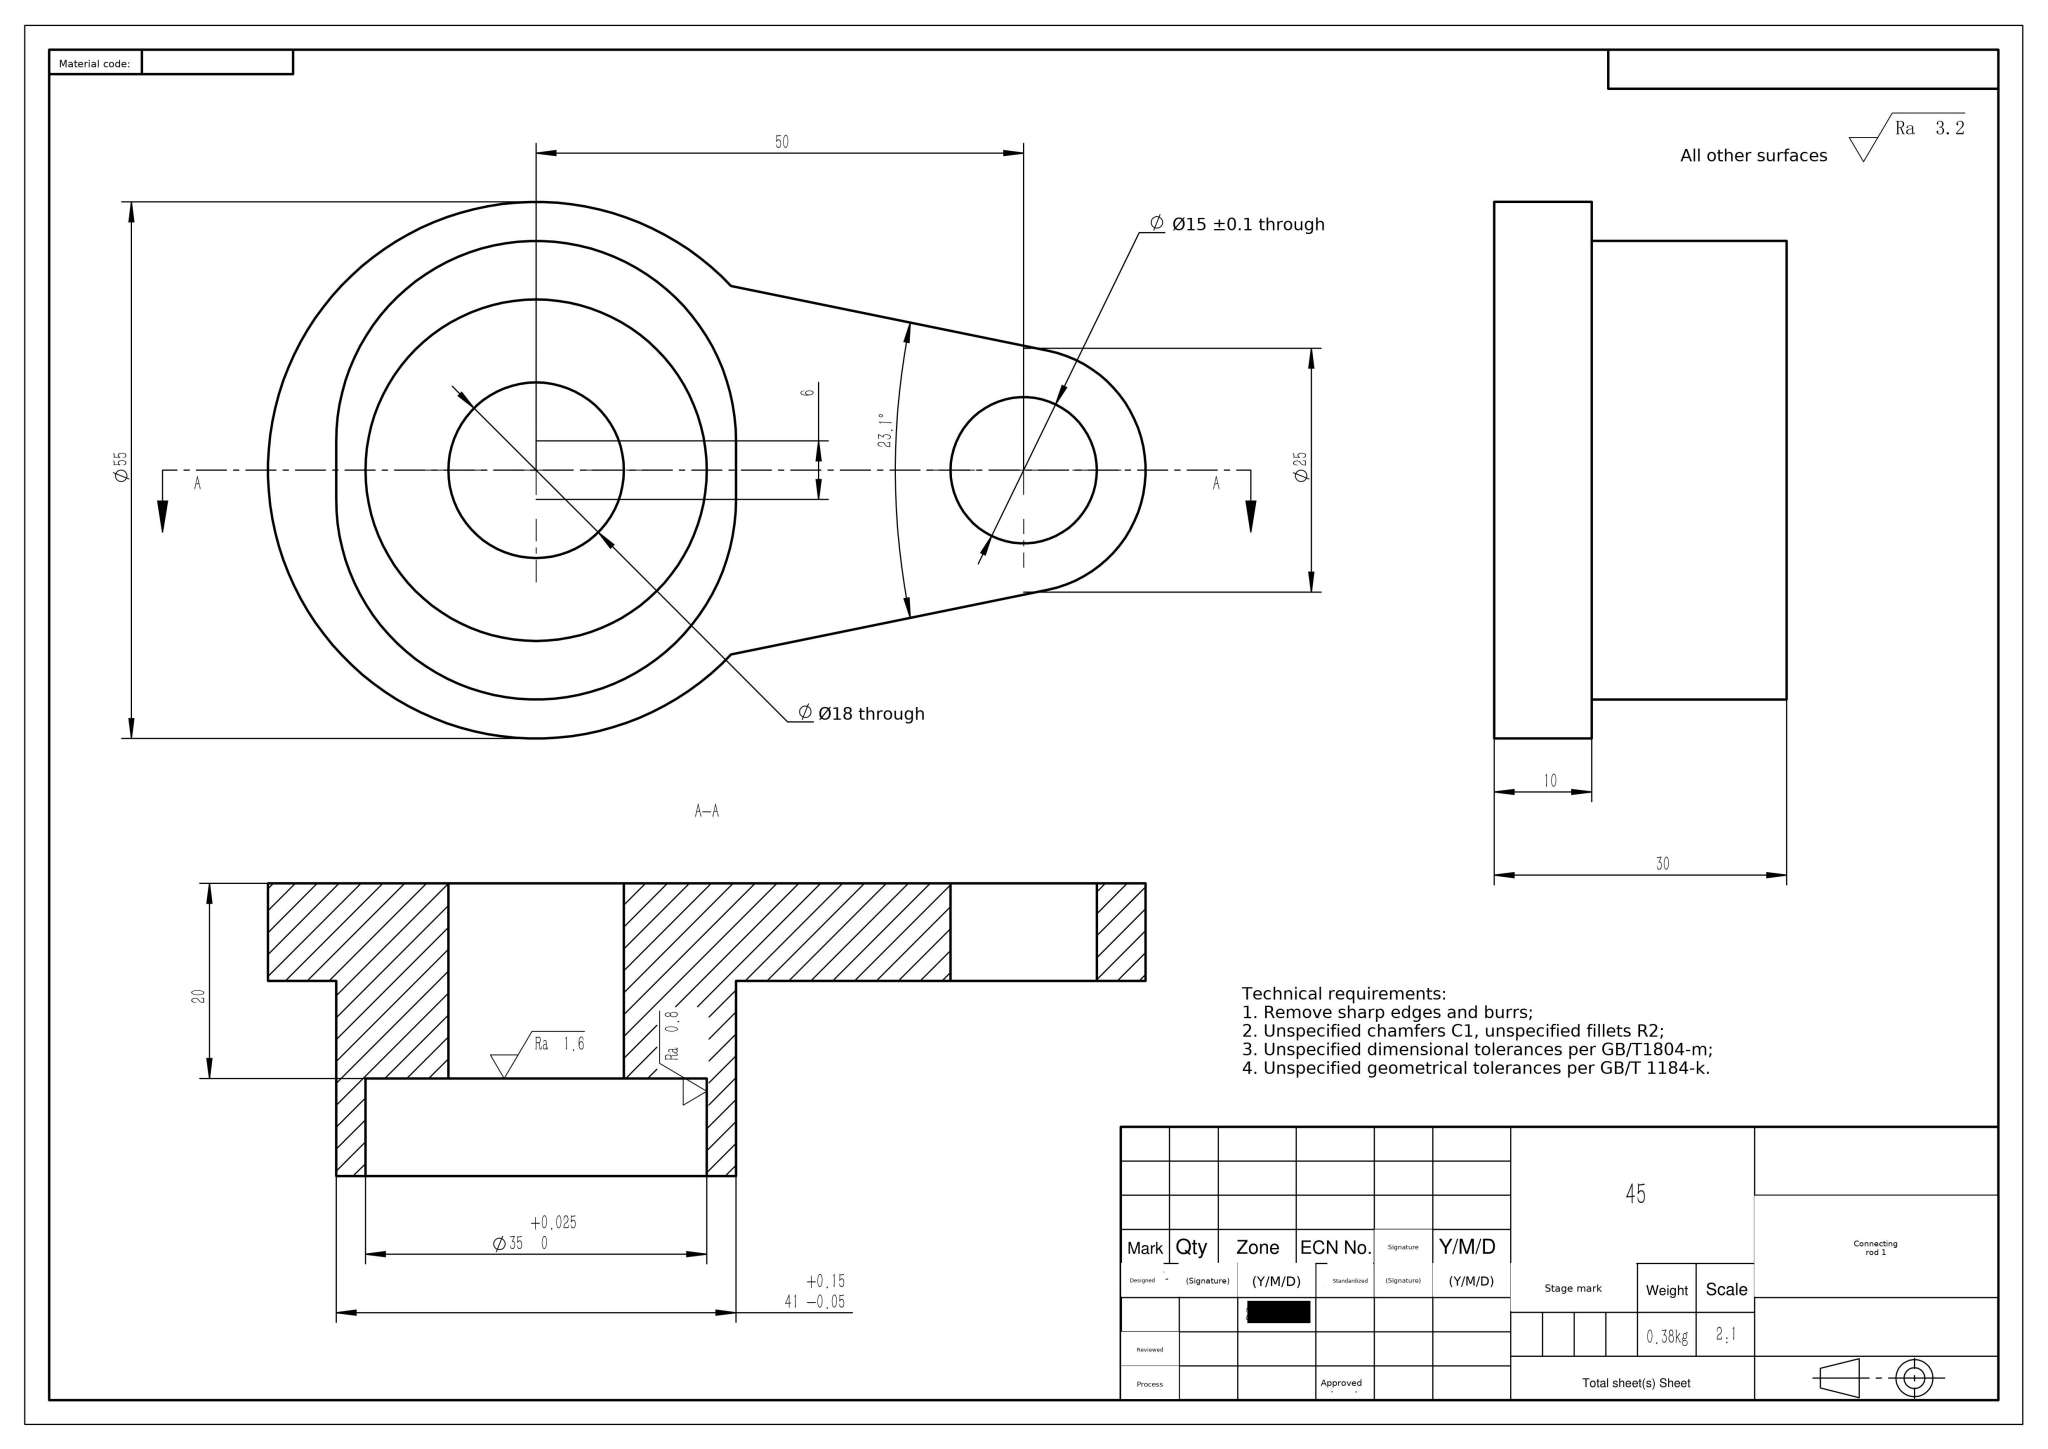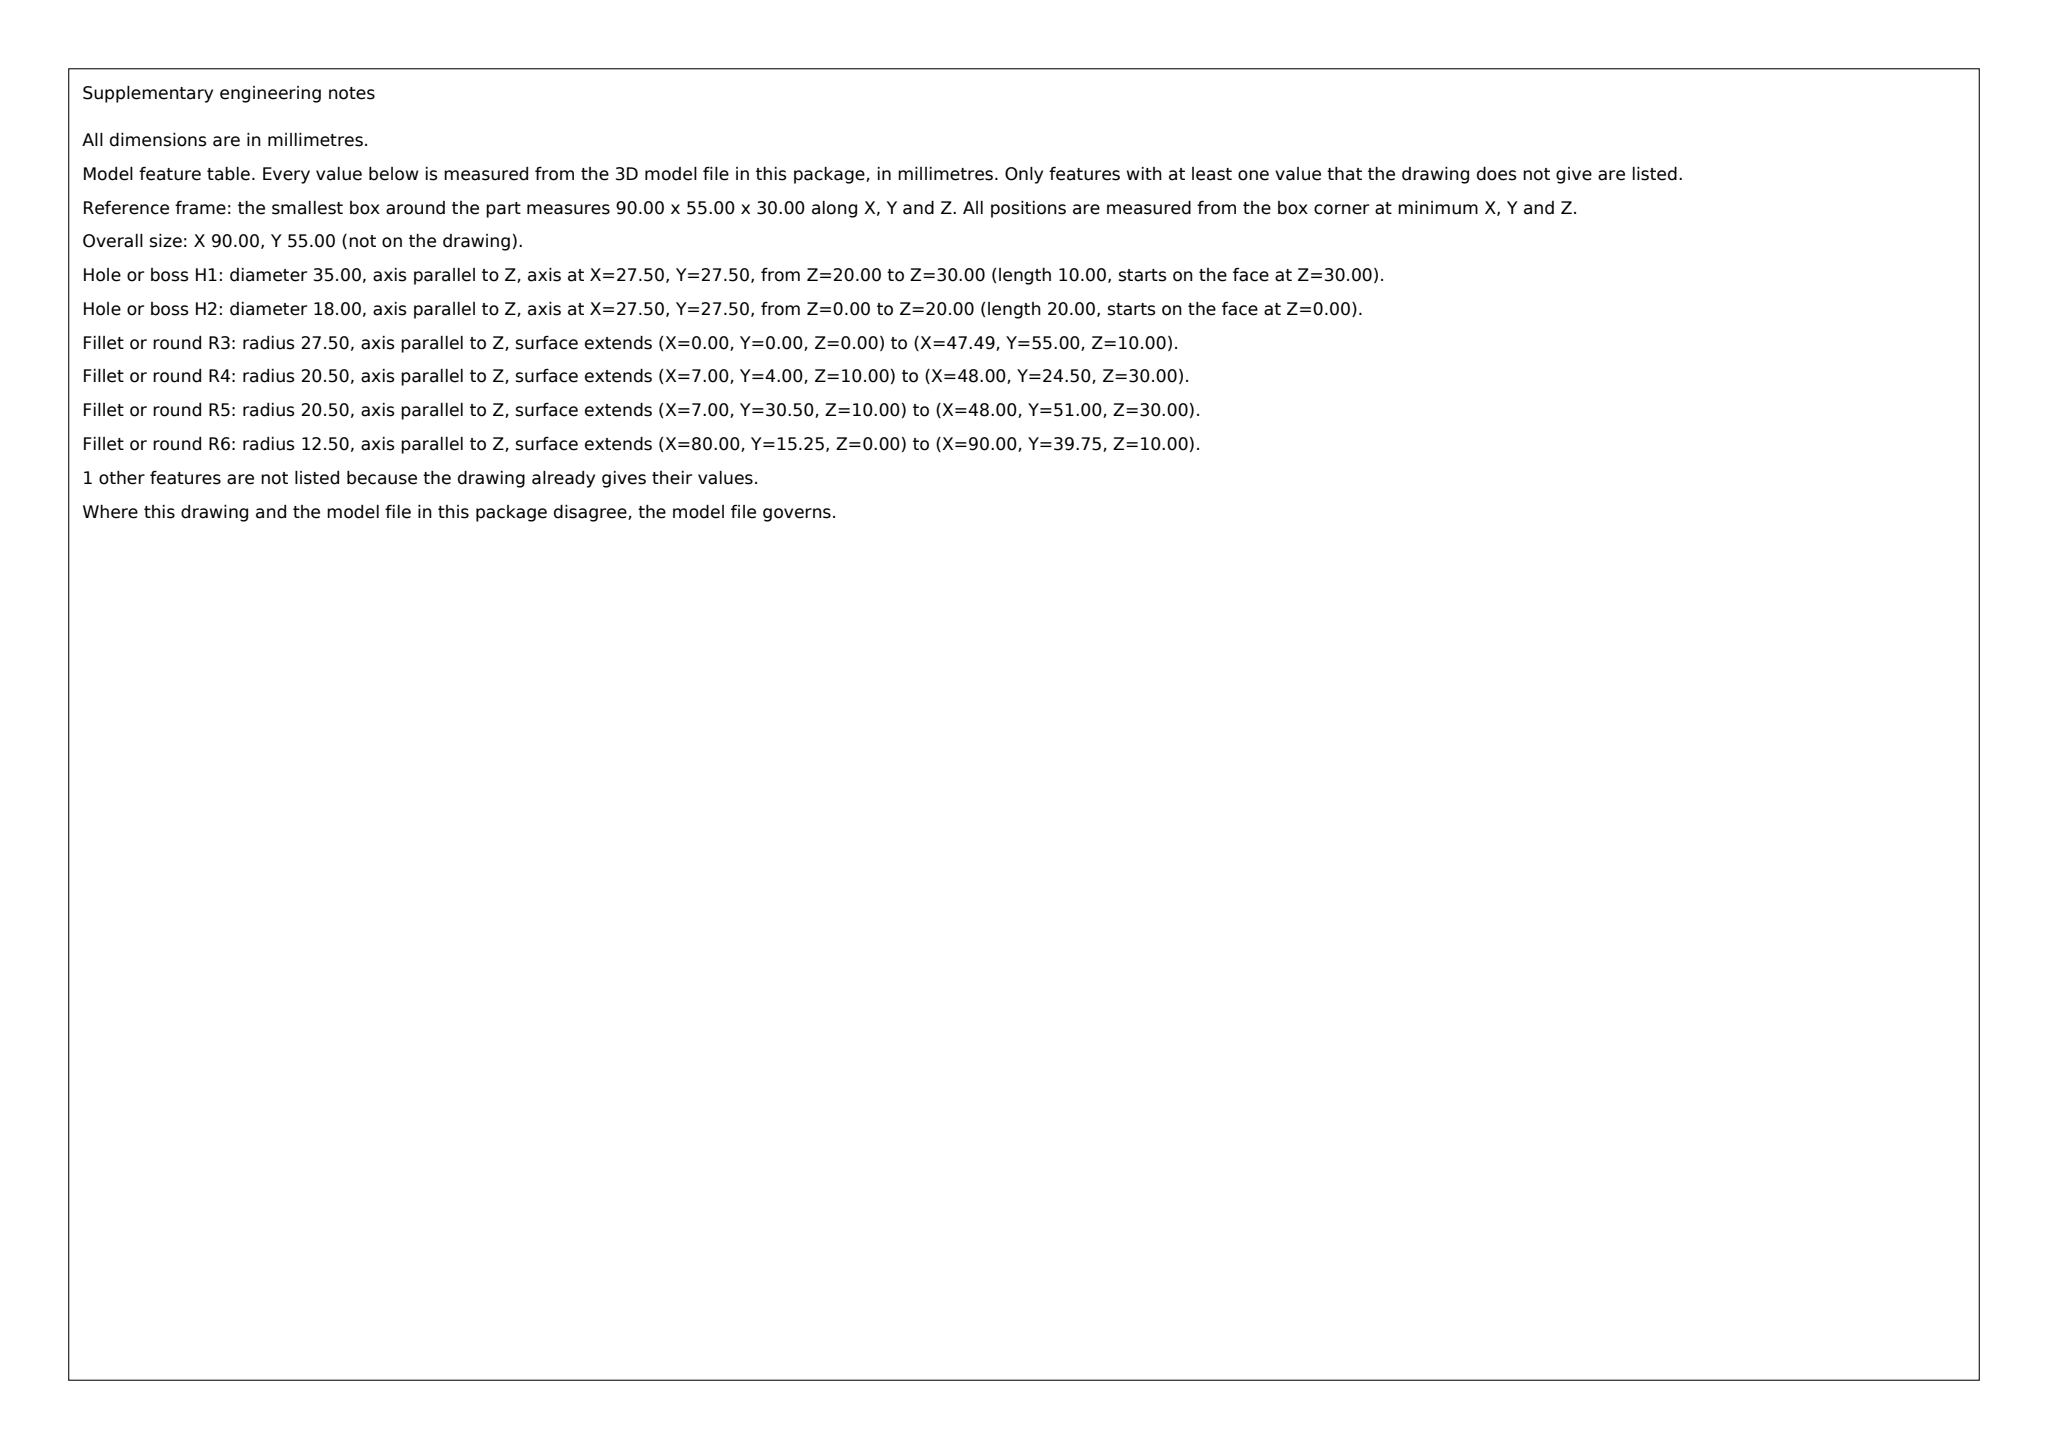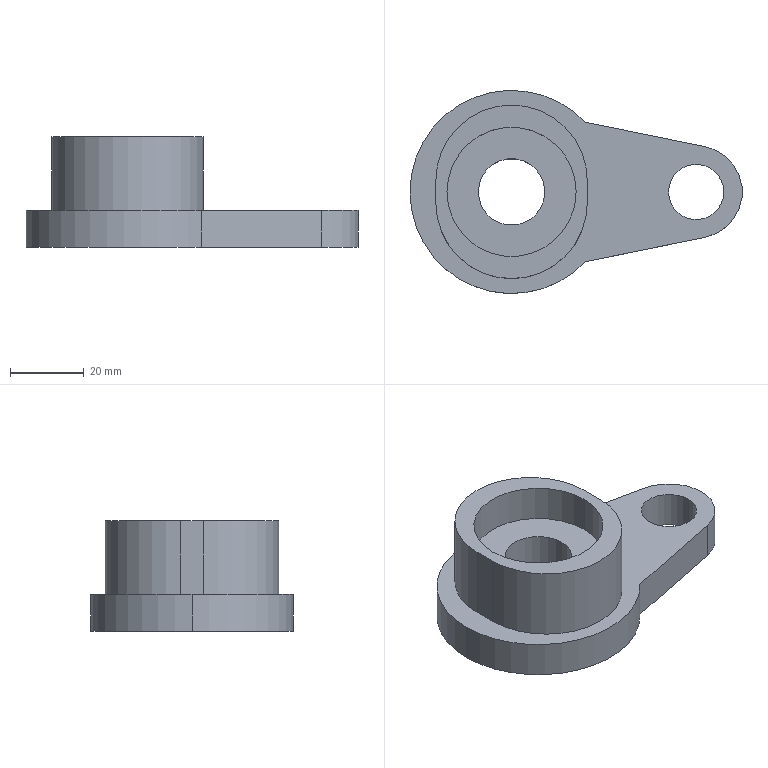Part | SolidWorks | mm | material 45 | 1 solid | 19 faces | box 90 x 55 x 30 mm | volume 48610 mm3 | cylinder 11 | plane 8 | commonest cylinder face diameters 15 x2 35 x2 55 x2 18 x2 41 x2 25 x1
build123d program:
from build123d import *

# Parameters (mm, degrees)
BOSS_EXTRUDE1_DEPTH     = 10
SKETCH5_R               = 27.5
BOSS_EXTRUDE3_DEPTH     = 10
BOSS_EXTRUDE4_DEPTH     = 20
CUT_EXTRUDE1_DEPTH      = 72.151
CUT_EXTRUDE1_DEPTH_BACK = 72.151
SKETCH2_R               = 9
CUT_EXTRUDE3_DEPTH      = 75.582
CUT_EXTRUDE3_DEPTH_BACK = 10
SKETCH7_R               = 17.5
SKETCH8_R               = 7.5
CUT_EXTRUDE4_DEPTH      = 72.151


with BuildPart() as part:
    # Sketch1 → Boss-Extrude1 (new body)
    with BuildSketch(Plane.XY):
        with BuildLine():
            Line((4.5, 22.045), (52.5, 12.247))
            ThreePointArc((52.5, 12.247), (62.5, 0), (52.5, -12.247))
            Line((52.5, -12.247), (4.5, -22.045))
            ThreePointArc((4.5, -22.045), (-22.5, 0), (4.5, 22.045))
        make_face()
    extrude(amount=BOSS_EXTRUDE1_DEPTH)

    # Sketch5 → Boss-Extrude3 (add)
    with BuildSketch(Plane(origin=(0, 0, 0), x_dir=(-1, 0, 0), z_dir=(0, 0, -1))):
        Circle(SKETCH5_R)
    extrude(amount=-BOSS_EXTRUDE3_DEPTH)

    # Sketch6 → Boss-Extrude4 (add)
    with BuildSketch(Plane.XY.offset(10)):
        with BuildLine():
            Line((-20.5, -3), (-20.5, 3))
            ThreePointArc((-20.5, 3), (0, 23.5), (20.5, 3))
            Line((20.5, 3), (20.5, -3))
            ThreePointArc((20.5, -3), (0, -23.5), (-20.5, -3))
        make_face()
    extrude(amount=BOSS_EXTRUDE4_DEPTH)

    # Sketch2 → Cut-Extrude1 (cut, two sides: drawn at the far end of the back side and taken through both)
    with BuildSketch(Plane.XY.offset(10).offset(-CUT_EXTRUDE1_DEPTH_BACK)):
        Circle(SKETCH2_R)
    extrude(amount=CUT_EXTRUDE1_DEPTH + CUT_EXTRUDE1_DEPTH_BACK, mode=Mode.SUBTRACT)

    # Sketch7 → Cut-Extrude3 (cut, two sides: drawn at the far end of the back side and taken through both)
    with BuildSketch(Plane.XY.offset(30).offset(-CUT_EXTRUDE3_DEPTH_BACK)):
        with Locations(Location((0, 0, 0), (0, 0, 180))):
            Circle(SKETCH7_R)
    extrude(amount=CUT_EXTRUDE3_DEPTH + CUT_EXTRUDE3_DEPTH_BACK, mode=Mode.SUBTRACT)

    # Sketch8 → Cut-Extrude4 (cut, through all)
    with BuildSketch(Plane.XY.offset(10)):
        with Locations((50, 0)):
            Circle(SKETCH8_R)
    extrude(amount=-CUT_EXTRUDE4_DEPTH, mode=Mode.SUBTRACT)


solid = part.part
STEP:
#1=CARTESIAN_POINT('',(42.5,0.,0.));
#2=VERTEX_POINT('',#1);
#3=CARTESIAN_POINT('',(57.5,0.,0.));
#4=VERTEX_POINT('',#3);
#5=CARTESIAN_POINT('',(50.,0.,0.));
#6=DIRECTION('',(0.,0.,1.));
#7=DIRECTION('',(1.,0.,0.));
#8=AXIS2_PLACEMENT_3D('',#5,#6,#7);
#9=CIRCLE('',#8,7.5);
#10=EDGE_CURVE('',#2,#4,#9,.T.);
#11=ORIENTED_EDGE('',*,*,#10,.F.);
#12=CARTESIAN_POINT('',(42.5,0.,10.));
#13=VERTEX_POINT('',#12);
#14=CARTESIAN_POINT('',(42.5,0.,0.));
#15=DIRECTION('',(0.,0.,1.));
#16=VECTOR('',#15,1000.);
#17=LINE('',#14,#16);
#18=EDGE_CURVE('',#2,#13,#17,.T.);
#19=ORIENTED_EDGE('',*,*,#18,.T.);
#20=CARTESIAN_POINT('',(57.5,0.,10.));
#21=VERTEX_POINT('',#20);
#22=CARTESIAN_POINT('',(50.,0.,10.));
#23=DIRECTION('',(0.,0.,1.));
#24=DIRECTION('',(1.,0.,0.));
#25=AXIS2_PLACEMENT_3D('',#22,#23,#24);
#26=CIRCLE('',#25,7.5);
#27=EDGE_CURVE('',#13,#21,#26,.T.);
#28=ORIENTED_EDGE('',*,*,#27,.T.);
#29=CARTESIAN_POINT('',(57.5,0.,0.));
#30=DIRECTION('',(0.,0.,1.));
#31=VECTOR('',#30,1000.);
#32=LINE('',#29,#31);
#33=EDGE_CURVE('',#4,#21,#32,.T.);
#34=ORIENTED_EDGE('',*,*,#33,.F.);
#35=EDGE_LOOP('',(#11,#19,#28,#34));
#36=FACE_OUTER_BOUND('',#35,.T.);
#37=CARTESIAN_POINT('',(50.,0.,0.));
#38=DIRECTION('',(0.,0.,1.));
#39=DIRECTION('',(1.,0.,0.));
#40=AXIS2_PLACEMENT_3D('',#37,#38,#39);
#41=CYLINDRICAL_SURFACE('',#40,7.5);
#42=ADVANCED_FACE('',(#36),#41,.F.);
#43=CARTESIAN_POINT('',(17.5,0.,30.));
#44=VERTEX_POINT('',#43);
#45=CARTESIAN_POINT('',(-17.5,0.,30.));
#46=VERTEX_POINT('',#45);
#47=CARTESIAN_POINT('',(0.,0.,30.));
#48=DIRECTION('',(0.,0.,-1.));
#49=DIRECTION('',(1.,0.,0.));
#50=AXIS2_PLACEMENT_3D('',#47,#48,#49);
#51=CIRCLE('',#50,17.5);
#52=EDGE_CURVE('',#44,#46,#51,.T.);
#53=ORIENTED_EDGE('',*,*,#52,.F.);
#54=CARTESIAN_POINT('',(17.5,0.,20.));
#55=VERTEX_POINT('',#54);
#56=CARTESIAN_POINT('',(17.5,0.,30.));
#57=DIRECTION('',(0.,0.,-1.));
#58=VECTOR('',#57,1000.);
#59=LINE('',#56,#58);
#60=EDGE_CURVE('',#44,#55,#59,.T.);
#61=ORIENTED_EDGE('',*,*,#60,.T.);
#62=CARTESIAN_POINT('',(-17.5,0.,20.));
#63=VERTEX_POINT('',#62);
#64=CARTESIAN_POINT('',(0.,0.,20.));
#65=DIRECTION('',(0.,0.,1.));
#66=DIRECTION('',(1.,0.,0.));
#67=AXIS2_PLACEMENT_3D('',#64,#65,#66);
#68=CIRCLE('',#67,17.5);
#69=EDGE_CURVE('',#63,#55,#68,.T.);
#70=ORIENTED_EDGE('',*,*,#69,.F.);
#71=CARTESIAN_POINT('',(-17.5,0.,30.));
#72=DIRECTION('',(0.,0.,-1.));
#73=VECTOR('',#72,1000.);
#74=LINE('',#71,#73);
#75=EDGE_CURVE('',#46,#63,#74,.T.);
#76=ORIENTED_EDGE('',*,*,#75,.F.);
#77=EDGE_LOOP('',(#53,#61,#70,#76));
#78=FACE_OUTER_BOUND('',#77,.T.);
#79=CARTESIAN_POINT('',(0.,0.,30.));
#80=DIRECTION('',(0.,0.,-1.));
#81=DIRECTION('',(-1.,0.,0.));
#82=AXIS2_PLACEMENT_3D('',#79,#80,#81);
#83=CYLINDRICAL_SURFACE('',#82,17.5);
#84=ADVANCED_FACE('',(#78),#83,.F.);
#85=CARTESIAN_POINT('',(19.992,-18.883,10.));
#86=VERTEX_POINT('',#85);
#87=CARTESIAN_POINT('',(-27.5,0.,10.));
#88=VERTEX_POINT('',#87);
#89=CARTESIAN_POINT('',(0.,0.,10.));
#90=DIRECTION('',(0.,0.,-1.));
#91=DIRECTION('',(-1.,0.,0.));
#92=AXIS2_PLACEMENT_3D('',#89,#90,#91);
#93=CIRCLE('',#92,27.5);
#94=EDGE_CURVE('',#86,#88,#93,.T.);
#95=ORIENTED_EDGE('',*,*,#94,.T.);
#96=CARTESIAN_POINT('',(-27.5,0.,0.));
#97=VERTEX_POINT('',#96);
#98=CARTESIAN_POINT('',(-27.5,0.,10.));
#99=DIRECTION('',(0.,0.,-1.));
#100=VECTOR('',#99,1000.);
#101=LINE('',#98,#100);
#102=EDGE_CURVE('',#88,#97,#101,.T.);
#103=ORIENTED_EDGE('',*,*,#102,.T.);
#104=CARTESIAN_POINT('',(19.992,-18.883,0.));
#105=VERTEX_POINT('',#104);
#106=CARTESIAN_POINT('',(0.,0.,0.));
#107=DIRECTION('',(0.,0.,-1.));
#108=DIRECTION('',(-1.,0.,0.));
#109=AXIS2_PLACEMENT_3D('',#106,#107,#108);
#110=CIRCLE('',#109,27.5);
#111=EDGE_CURVE('',#105,#97,#110,.T.);
#112=ORIENTED_EDGE('',*,*,#111,.F.);
#113=CARTESIAN_POINT('',(19.992,-18.883,10.));
#114=DIRECTION('',(0.,0.,-1.));
#115=VECTOR('',#114,1000.);
#116=LINE('',#113,#115);
#117=EDGE_CURVE('',#86,#105,#116,.T.);
#118=ORIENTED_EDGE('',*,*,#117,.F.);
#119=EDGE_LOOP('',(#95,#103,#112,#118));
#120=FACE_OUTER_BOUND('',#119,.T.);
#121=CARTESIAN_POINT('',(0.,0.,10.));
#122=DIRECTION('',(0.,0.,-1.));
#123=DIRECTION('',(-1.,0.,0.));
#124=AXIS2_PLACEMENT_3D('',#121,#122,#123);
#125=CYLINDRICAL_SURFACE('',#124,27.5);
#126=ADVANCED_FACE('',(#120),#125,.T.);
#127=CARTESIAN_POINT('',(-9.,0.,0.));
#128=VERTEX_POINT('',#127);
#129=CARTESIAN_POINT('',(9.,0.,0.));
#130=VERTEX_POINT('',#129);
#131=CARTESIAN_POINT('',(0.,0.,0.));
#132=DIRECTION('',(0.,0.,1.));
#133=DIRECTION('',(1.,0.,0.));
#134=AXIS2_PLACEMENT_3D('',#131,#132,#133);
#135=CIRCLE('',#134,9.);
#136=EDGE_CURVE('',#128,#130,#135,.T.);
#137=ORIENTED_EDGE('',*,*,#136,.F.);
#138=CARTESIAN_POINT('',(-9.,0.,20.));
#139=VERTEX_POINT('',#138);
#140=CARTESIAN_POINT('',(-9.,0.,0.));
#141=DIRECTION('',(0.,0.,1.));
#142=VECTOR('',#141,1000.);
#143=LINE('',#140,#142);
#144=EDGE_CURVE('',#128,#139,#143,.T.);
#145=ORIENTED_EDGE('',*,*,#144,.T.);
#146=CARTESIAN_POINT('',(9.,0.,20.));
#147=VERTEX_POINT('',#146);
#148=CARTESIAN_POINT('',(0.,0.,20.));
#149=DIRECTION('',(0.,0.,-1.));
#150=DIRECTION('',(1.,0.,0.));
#151=AXIS2_PLACEMENT_3D('',#148,#149,#150);
#152=CIRCLE('',#151,9.);
#153=EDGE_CURVE('',#147,#139,#152,.T.);
#154=ORIENTED_EDGE('',*,*,#153,.F.);
#155=CARTESIAN_POINT('',(9.,0.,0.));
#156=DIRECTION('',(0.,0.,1.));
#157=VECTOR('',#156,1000.);
#158=LINE('',#155,#157);
#159=EDGE_CURVE('',#130,#147,#158,.T.);
#160=ORIENTED_EDGE('',*,*,#159,.F.);
#161=EDGE_LOOP('',(#137,#145,#154,#160));
#162=FACE_OUTER_BOUND('',#161,.T.);
#163=CARTESIAN_POINT('',(0.,0.,0.));
#164=DIRECTION('',(0.,0.,1.));
#165=DIRECTION('',(1.,0.,0.));
#166=AXIS2_PLACEMENT_3D('',#163,#164,#165);
#167=CYLINDRICAL_SURFACE('',#166,9.);
#168=ADVANCED_FACE('',(#162),#167,.F.);
#169=ORIENTED_EDGE('',*,*,#144,.F.);
#170=CARTESIAN_POINT('',(0.,0.,0.));
#171=DIRECTION('',(0.,0.,1.));
#172=DIRECTION('',(1.,0.,0.));
#173=AXIS2_PLACEMENT_3D('',#170,#171,#172);
#174=CIRCLE('',#173,9.);
#175=EDGE_CURVE('',#130,#128,#174,.T.);
#176=ORIENTED_EDGE('',*,*,#175,.F.);
#177=ORIENTED_EDGE('',*,*,#159,.T.);
#178=CARTESIAN_POINT('',(0.,0.,20.));
#179=DIRECTION('',(0.,0.,-1.));
#180=DIRECTION('',(1.,0.,0.));
#181=AXIS2_PLACEMENT_3D('',#178,#179,#180);
#182=CIRCLE('',#181,9.);
#183=EDGE_CURVE('',#139,#147,#182,.T.);
#184=ORIENTED_EDGE('',*,*,#183,.F.);
#185=EDGE_LOOP('',(#169,#176,#177,#184));
#186=FACE_OUTER_BOUND('',#185,.T.);
#187=CARTESIAN_POINT('',(0.,0.,0.));
#188=DIRECTION('',(0.,0.,1.));
#189=DIRECTION('',(1.,0.,0.));
#190=AXIS2_PLACEMENT_3D('',#187,#188,#189);
#191=CYLINDRICAL_SURFACE('',#190,9.);
#192=ADVANCED_FACE('',(#186),#191,.F.);
#193=CARTESIAN_POINT('',(52.5,-12.247,10.));
#194=VERTEX_POINT('',#193);
#195=CARTESIAN_POINT('',(52.5,-12.247,10.));
#196=DIRECTION('',(0.9798,0.2,0.));
#197=VECTOR('',#196,1000.);
#198=LINE('',#195,#197);
#199=EDGE_CURVE('',#86,#194,#198,.T.);
#200=ORIENTED_EDGE('',*,*,#199,.F.);
#201=ORIENTED_EDGE('',*,*,#117,.T.);
#202=CARTESIAN_POINT('',(52.5,-12.247,0.));
#203=VERTEX_POINT('',#202);
#204=CARTESIAN_POINT('',(52.5,-12.247,0.));
#205=DIRECTION('',(0.9798,0.2,0.));
#206=VECTOR('',#205,1000.);
#207=LINE('',#204,#206);
#208=EDGE_CURVE('',#105,#203,#207,.T.);
#209=ORIENTED_EDGE('',*,*,#208,.T.);
#210=CARTESIAN_POINT('',(52.5,-12.247,10.));
#211=DIRECTION('',(0.,0.,-1.));
#212=VECTOR('',#211,1000.);
#213=LINE('',#210,#212);
#214=EDGE_CURVE('',#194,#203,#213,.T.);
#215=ORIENTED_EDGE('',*,*,#214,.F.);
#216=EDGE_LOOP('',(#200,#201,#209,#215));
#217=FACE_OUTER_BOUND('',#216,.T.);
#218=CARTESIAN_POINT('',(52.5,-12.247,10.));
#219=DIRECTION('',(-0.2,0.9798,0.));
#220=DIRECTION('',(-0.9798,-0.2,0.));
#221=AXIS2_PLACEMENT_3D('',#218,#219,#220);
#222=PLANE('',#221);
#223=ADVANCED_FACE('',(#217),#222,.F.);
#224=CARTESIAN_POINT('',(52.5,12.247,0.));
#225=VERTEX_POINT('',#224);
#226=CARTESIAN_POINT('',(50.,0.,0.));
#227=DIRECTION('',(0.,0.,1.));
#228=DIRECTION('',(-1.,0.,0.));
#229=AXIS2_PLACEMENT_3D('',#226,#227,#228);
#230=CIRCLE('',#229,12.5);
#231=EDGE_CURVE('',#203,#225,#230,.T.);
#232=ORIENTED_EDGE('',*,*,#231,.T.);
#233=CARTESIAN_POINT('',(52.5,12.247,10.));
#234=VERTEX_POINT('',#233);
#235=CARTESIAN_POINT('',(52.5,12.247,10.));
#236=DIRECTION('',(0.,0.,-1.));
#237=VECTOR('',#236,1000.);
#238=LINE('',#235,#237);
#239=EDGE_CURVE('',#234,#225,#238,.T.);
#240=ORIENTED_EDGE('',*,*,#239,.F.);
#241=CARTESIAN_POINT('',(50.,0.,10.));
#242=DIRECTION('',(0.,0.,1.));
#243=DIRECTION('',(-1.,0.,0.));
#244=AXIS2_PLACEMENT_3D('',#241,#242,#243);
#245=CIRCLE('',#244,12.5);
#246=EDGE_CURVE('',#194,#234,#245,.T.);
#247=ORIENTED_EDGE('',*,*,#246,.F.);
#248=ORIENTED_EDGE('',*,*,#214,.T.);
#249=EDGE_LOOP('',(#232,#240,#247,#248));
#250=FACE_OUTER_BOUND('',#249,.T.);
#251=CARTESIAN_POINT('',(50.,0.,10.));
#252=DIRECTION('',(0.,0.,-1.));
#253=DIRECTION('',(-1.,0.,0.));
#254=AXIS2_PLACEMENT_3D('',#251,#252,#253);
#255=CYLINDRICAL_SURFACE('',#254,12.5);
#256=ADVANCED_FACE('',(#250),#255,.T.);
#257=CARTESIAN_POINT('',(19.992,18.883,0.));
#258=VERTEX_POINT('',#257);
#259=CARTESIAN_POINT('',(4.5,22.045,0.));
#260=DIRECTION('',(-0.9798,0.2,0.));
#261=VECTOR('',#260,1000.);
#262=LINE('',#259,#261);
#263=EDGE_CURVE('',#225,#258,#262,.T.);
#264=ORIENTED_EDGE('',*,*,#263,.T.);
#265=CARTESIAN_POINT('',(19.992,18.883,10.));
#266=VERTEX_POINT('',#265);
#267=CARTESIAN_POINT('',(19.992,18.883,10.));
#268=DIRECTION('',(0.,0.,1.));
#269=VECTOR('',#268,1000.);
#270=LINE('',#267,#269);
#271=EDGE_CURVE('',#258,#266,#270,.T.);
#272=ORIENTED_EDGE('',*,*,#271,.T.);
#273=CARTESIAN_POINT('',(4.5,22.045,10.));
#274=DIRECTION('',(-0.9798,0.2,0.));
#275=VECTOR('',#274,1000.);
#276=LINE('',#273,#275);
#277=EDGE_CURVE('',#234,#266,#276,.T.);
#278=ORIENTED_EDGE('',*,*,#277,.F.);
#279=ORIENTED_EDGE('',*,*,#239,.T.);
#280=EDGE_LOOP('',(#264,#272,#278,#279));
#281=FACE_OUTER_BOUND('',#280,.T.);
#282=CARTESIAN_POINT('',(4.5,22.045,10.));
#283=DIRECTION('',(-0.2,-0.9798,0.));
#284=DIRECTION('',(0.9798,-0.2,0.));
#285=AXIS2_PLACEMENT_3D('',#282,#283,#284);
#286=PLANE('',#285);
#287=ADVANCED_FACE('',(#281),#286,.F.);
#288=CARTESIAN_POINT('',(50.,0.,10.));
#289=DIRECTION('',(0.,0.,1.));
#290=DIRECTION('',(1.,0.,0.));
#291=AXIS2_PLACEMENT_3D('',#288,#289,#290);
#292=CIRCLE('',#291,7.5);
#293=EDGE_CURVE('',#21,#13,#292,.T.);
#294=ORIENTED_EDGE('',*,*,#293,.F.);
#295=ORIENTED_EDGE('',*,*,#27,.F.);
#296=EDGE_LOOP('',(#294,#295));
#297=FACE_BOUND('',#296,.T.);
#298=CARTESIAN_POINT('',(-20.5,-3.,10.));
#299=VERTEX_POINT('',#298);
#300=CARTESIAN_POINT('',(20.5,-3.,10.));
#301=VERTEX_POINT('',#300);
#302=CARTESIAN_POINT('',(0.,-3.,10.));
#303=DIRECTION('',(0.,0.,1.));
#304=DIRECTION('',(1.,0.,0.));
#305=AXIS2_PLACEMENT_3D('',#302,#303,#304);
#306=CIRCLE('',#305,20.5);
#307=EDGE_CURVE('',#299,#301,#306,.T.);
#308=ORIENTED_EDGE('',*,*,#307,.F.);
#309=CARTESIAN_POINT('',(-20.5,3.,10.));
#310=VERTEX_POINT('',#309);
#311=CARTESIAN_POINT('',(-20.5,-3.,10.));
#312=DIRECTION('',(0.,-1.,0.));
#313=VECTOR('',#312,1000.);
#314=LINE('',#311,#313);
#315=EDGE_CURVE('',#310,#299,#314,.T.);
#316=ORIENTED_EDGE('',*,*,#315,.F.);
#317=CARTESIAN_POINT('',(20.5,3.,10.));
#318=VERTEX_POINT('',#317);
#319=CARTESIAN_POINT('',(-0.,3.,10.));
#320=DIRECTION('',(0.,0.,1.));
#321=DIRECTION('',(1.,0.,0.));
#322=AXIS2_PLACEMENT_3D('',#319,#320,#321);
#323=CIRCLE('',#322,20.5);
#324=EDGE_CURVE('',#318,#310,#323,.T.);
#325=ORIENTED_EDGE('',*,*,#324,.F.);
#326=CARTESIAN_POINT('',(20.5,-3.,10.));
#327=DIRECTION('',(0.,1.,0.));
#328=VECTOR('',#327,1000.);
#329=LINE('',#326,#328);
#330=EDGE_CURVE('',#301,#318,#329,.T.);
#331=ORIENTED_EDGE('',*,*,#330,.F.);
#332=EDGE_LOOP('',(#308,#316,#325,#331));
#333=FACE_BOUND('',#332,.T.);
#334=ORIENTED_EDGE('',*,*,#94,.F.);
#335=ORIENTED_EDGE('',*,*,#199,.T.);
#336=ORIENTED_EDGE('',*,*,#246,.T.);
#337=ORIENTED_EDGE('',*,*,#277,.T.);
#338=CARTESIAN_POINT('',(0.,0.,10.));
#339=DIRECTION('',(0.,0.,-1.));
#340=DIRECTION('',(-1.,0.,0.));
#341=AXIS2_PLACEMENT_3D('',#338,#339,#340);
#342=CIRCLE('',#341,27.5);
#343=EDGE_CURVE('',#88,#266,#342,.T.);
#344=ORIENTED_EDGE('',*,*,#343,.F.);
#345=EDGE_LOOP('',(#334,#335,#336,#337,#344));
#346=FACE_OUTER_BOUND('',#345,.T.);
#347=CARTESIAN_POINT('',(0.,0.,10.));
#348=DIRECTION('',(0.,0.,1.));
#349=DIRECTION('',(1.,0.,0.));
#350=AXIS2_PLACEMENT_3D('',#347,#348,#349);
#351=PLANE('',#350);
#352=ADVANCED_FACE('',(#297,#333,#346),#351,.T.);
#353=CARTESIAN_POINT('',(50.,0.,0.));
#354=DIRECTION('',(0.,0.,1.));
#355=DIRECTION('',(1.,0.,0.));
#356=AXIS2_PLACEMENT_3D('',#353,#354,#355);
#357=CIRCLE('',#356,7.5);
#358=EDGE_CURVE('',#4,#2,#357,.T.);
#359=ORIENTED_EDGE('',*,*,#358,.T.);
#360=ORIENTED_EDGE('',*,*,#10,.T.);
#361=EDGE_LOOP('',(#359,#360));
#362=FACE_BOUND('',#361,.T.);
#363=ORIENTED_EDGE('',*,*,#175,.T.);
#364=ORIENTED_EDGE('',*,*,#136,.T.);
#365=EDGE_LOOP('',(#363,#364));
#366=FACE_BOUND('',#365,.T.);
#367=ORIENTED_EDGE('',*,*,#208,.F.);
#368=ORIENTED_EDGE('',*,*,#111,.T.);
#369=CARTESIAN_POINT('',(0.,0.,0.));
#370=DIRECTION('',(0.,0.,-1.));
#371=DIRECTION('',(-1.,0.,0.));
#372=AXIS2_PLACEMENT_3D('',#369,#370,#371);
#373=CIRCLE('',#372,27.5);
#374=EDGE_CURVE('',#97,#258,#373,.T.);
#375=ORIENTED_EDGE('',*,*,#374,.T.);
#376=ORIENTED_EDGE('',*,*,#263,.F.);
#377=ORIENTED_EDGE('',*,*,#231,.F.);
#378=EDGE_LOOP('',(#367,#368,#375,#376,#377));
#379=FACE_OUTER_BOUND('',#378,.T.);
#380=CARTESIAN_POINT('',(0.,0.,0.));
#381=DIRECTION('',(0.,0.,1.));
#382=DIRECTION('',(1.,0.,0.));
#383=AXIS2_PLACEMENT_3D('',#380,#381,#382);
#384=PLANE('',#383);
#385=ADVANCED_FACE('',(#362,#366,#379),#384,.F.);
#386=ORIENTED_EDGE('',*,*,#102,.F.);
#387=ORIENTED_EDGE('',*,*,#343,.T.);
#388=ORIENTED_EDGE('',*,*,#271,.F.);
#389=ORIENTED_EDGE('',*,*,#374,.F.);
#390=EDGE_LOOP('',(#386,#387,#388,#389));
#391=FACE_OUTER_BOUND('',#390,.T.);
#392=CARTESIAN_POINT('',(0.,0.,10.));
#393=DIRECTION('',(0.,0.,-1.));
#394=DIRECTION('',(-1.,0.,0.));
#395=AXIS2_PLACEMENT_3D('',#392,#393,#394);
#396=CYLINDRICAL_SURFACE('',#395,27.5);
#397=ADVANCED_FACE('',(#391),#396,.T.);
#398=ORIENTED_EDGE('',*,*,#307,.T.);
#399=CARTESIAN_POINT('',(20.5,-3.,30.));
#400=VERTEX_POINT('',#399);
#401=CARTESIAN_POINT('',(20.5,-3.,30.));
#402=DIRECTION('',(0.,0.,-1.));
#403=VECTOR('',#402,1000.);
#404=LINE('',#401,#403);
#405=EDGE_CURVE('',#400,#301,#404,.T.);
#406=ORIENTED_EDGE('',*,*,#405,.F.);
#407=CARTESIAN_POINT('',(-20.5,-3.,30.));
#408=VERTEX_POINT('',#407);
#409=CARTESIAN_POINT('',(0.,-3.,30.));
#410=DIRECTION('',(0.,0.,1.));
#411=DIRECTION('',(1.,0.,0.));
#412=AXIS2_PLACEMENT_3D('',#409,#410,#411);
#413=CIRCLE('',#412,20.5);
#414=EDGE_CURVE('',#408,#400,#413,.T.);
#415=ORIENTED_EDGE('',*,*,#414,.F.);
#416=CARTESIAN_POINT('',(-20.5,-3.,30.));
#417=DIRECTION('',(0.,0.,-1.));
#418=VECTOR('',#417,1000.);
#419=LINE('',#416,#418);
#420=EDGE_CURVE('',#408,#299,#419,.T.);
#421=ORIENTED_EDGE('',*,*,#420,.T.);
#422=EDGE_LOOP('',(#398,#406,#415,#421));
#423=FACE_OUTER_BOUND('',#422,.T.);
#424=CARTESIAN_POINT('',(0.,-3.,30.));
#425=DIRECTION('',(0.,0.,-1.));
#426=DIRECTION('',(-1.,0.,0.));
#427=AXIS2_PLACEMENT_3D('',#424,#425,#426);
#428=CYLINDRICAL_SURFACE('',#427,20.5);
#429=ADVANCED_FACE('',(#423),#428,.T.);
#430=ORIENTED_EDGE('',*,*,#330,.T.);
#431=CARTESIAN_POINT('',(20.5,3.,30.));
#432=VERTEX_POINT('',#431);
#433=CARTESIAN_POINT('',(20.5,3.,30.));
#434=DIRECTION('',(0.,0.,-1.));
#435=VECTOR('',#434,1000.);
#436=LINE('',#433,#435);
#437=EDGE_CURVE('',#432,#318,#436,.T.);
#438=ORIENTED_EDGE('',*,*,#437,.F.);
#439=CARTESIAN_POINT('',(20.5,-3.,30.));
#440=DIRECTION('',(0.,1.,0.));
#441=VECTOR('',#440,1000.);
#442=LINE('',#439,#441);
#443=EDGE_CURVE('',#400,#432,#442,.T.);
#444=ORIENTED_EDGE('',*,*,#443,.F.);
#445=ORIENTED_EDGE('',*,*,#405,.T.);
#446=EDGE_LOOP('',(#430,#438,#444,#445));
#447=FACE_OUTER_BOUND('',#446,.T.);
#448=CARTESIAN_POINT('',(20.5,-3.,30.));
#449=DIRECTION('',(-1.,0.,0.));
#450=DIRECTION('',(0.,0.,1.));
#451=AXIS2_PLACEMENT_3D('',#448,#449,#450);
#452=PLANE('',#451);
#453=ADVANCED_FACE('',(#447),#452,.F.);
#454=ORIENTED_EDGE('',*,*,#324,.T.);
#455=CARTESIAN_POINT('',(-20.5,3.,30.));
#456=VERTEX_POINT('',#455);
#457=CARTESIAN_POINT('',(-20.5,3.,30.));
#458=DIRECTION('',(0.,0.,-1.));
#459=VECTOR('',#458,1000.);
#460=LINE('',#457,#459);
#461=EDGE_CURVE('',#456,#310,#460,.T.);
#462=ORIENTED_EDGE('',*,*,#461,.F.);
#463=CARTESIAN_POINT('',(-0.,3.,30.));
#464=DIRECTION('',(0.,0.,1.));
#465=DIRECTION('',(1.,0.,0.));
#466=AXIS2_PLACEMENT_3D('',#463,#464,#465);
#467=CIRCLE('',#466,20.5);
#468=EDGE_CURVE('',#432,#456,#467,.T.);
#469=ORIENTED_EDGE('',*,*,#468,.F.);
#470=ORIENTED_EDGE('',*,*,#437,.T.);
#471=EDGE_LOOP('',(#454,#462,#469,#470));
#472=FACE_OUTER_BOUND('',#471,.T.);
#473=CARTESIAN_POINT('',(-0.,3.,30.));
#474=DIRECTION('',(0.,0.,-1.));
#475=DIRECTION('',(-1.,0.,0.));
#476=AXIS2_PLACEMENT_3D('',#473,#474,#475);
#477=CYLINDRICAL_SURFACE('',#476,20.5);
#478=ADVANCED_FACE('',(#472),#477,.T.);
#479=ORIENTED_EDGE('',*,*,#315,.T.);
#480=ORIENTED_EDGE('',*,*,#420,.F.);
#481=CARTESIAN_POINT('',(-20.5,-3.,30.));
#482=DIRECTION('',(0.,-1.,0.));
#483=VECTOR('',#482,1000.);
#484=LINE('',#481,#483);
#485=EDGE_CURVE('',#456,#408,#484,.T.);
#486=ORIENTED_EDGE('',*,*,#485,.F.);
#487=ORIENTED_EDGE('',*,*,#461,.T.);
#488=EDGE_LOOP('',(#479,#480,#486,#487));
#489=FACE_OUTER_BOUND('',#488,.T.);
#490=CARTESIAN_POINT('',(-20.5,-3.,30.));
#491=DIRECTION('',(1.,0.,0.));
#492=DIRECTION('',(0.,0.,-1.));
#493=AXIS2_PLACEMENT_3D('',#490,#491,#492);
#494=PLANE('',#493);
#495=ADVANCED_FACE('',(#489),#494,.F.);
#496=CARTESIAN_POINT('',(0.,0.,30.));
#497=DIRECTION('',(0.,0.,-1.));
#498=DIRECTION('',(1.,0.,0.));
#499=AXIS2_PLACEMENT_3D('',#496,#497,#498);
#500=CIRCLE('',#499,17.5);
#501=EDGE_CURVE('',#46,#44,#500,.T.);
#502=ORIENTED_EDGE('',*,*,#501,.T.);
#503=ORIENTED_EDGE('',*,*,#52,.T.);
#504=EDGE_LOOP('',(#502,#503));
#505=FACE_BOUND('',#504,.T.);
#506=ORIENTED_EDGE('',*,*,#414,.T.);
#507=ORIENTED_EDGE('',*,*,#443,.T.);
#508=ORIENTED_EDGE('',*,*,#468,.T.);
#509=ORIENTED_EDGE('',*,*,#485,.T.);
#510=EDGE_LOOP('',(#506,#507,#508,#509));
#511=FACE_OUTER_BOUND('',#510,.T.);
#512=CARTESIAN_POINT('',(0.,-3.,30.));
#513=DIRECTION('',(0.,0.,1.));
#514=DIRECTION('',(1.,0.,0.));
#515=AXIS2_PLACEMENT_3D('',#512,#513,#514);
#516=PLANE('',#515);
#517=ADVANCED_FACE('',(#505,#511),#516,.T.);
#518=ORIENTED_EDGE('',*,*,#69,.T.);
#519=CARTESIAN_POINT('',(0.,0.,20.));
#520=DIRECTION('',(0.,0.,1.));
#521=DIRECTION('',(1.,0.,0.));
#522=AXIS2_PLACEMENT_3D('',#519,#520,#521);
#523=CIRCLE('',#522,17.5);
#524=EDGE_CURVE('',#55,#63,#523,.T.);
#525=ORIENTED_EDGE('',*,*,#524,.T.);
#526=EDGE_LOOP('',(#518,#525));
#527=FACE_OUTER_BOUND('',#526,.T.);
#528=ORIENTED_EDGE('',*,*,#153,.T.);
#529=ORIENTED_EDGE('',*,*,#183,.T.);
#530=EDGE_LOOP('',(#528,#529));
#531=FACE_BOUND('',#530,.T.);
#532=CARTESIAN_POINT('',(0.,0.,20.));
#533=DIRECTION('',(0.,0.,1.));
#534=DIRECTION('',(1.,0.,0.));
#535=AXIS2_PLACEMENT_3D('',#532,#533,#534);
#536=PLANE('',#535);
#537=ADVANCED_FACE('',(#527,#531),#536,.T.);
#538=ORIENTED_EDGE('',*,*,#60,.F.);
#539=ORIENTED_EDGE('',*,*,#501,.F.);
#540=ORIENTED_EDGE('',*,*,#75,.T.);
#541=ORIENTED_EDGE('',*,*,#524,.F.);
#542=EDGE_LOOP('',(#538,#539,#540,#541));
#543=FACE_OUTER_BOUND('',#542,.T.);
#544=CARTESIAN_POINT('',(0.,0.,30.));
#545=DIRECTION('',(0.,0.,-1.));
#546=DIRECTION('',(-1.,0.,0.));
#547=AXIS2_PLACEMENT_3D('',#544,#545,#546);
#548=CYLINDRICAL_SURFACE('',#547,17.5);
#549=ADVANCED_FACE('',(#543),#548,.F.);
#550=ORIENTED_EDGE('',*,*,#18,.F.);
#551=ORIENTED_EDGE('',*,*,#358,.F.);
#552=ORIENTED_EDGE('',*,*,#33,.T.);
#553=ORIENTED_EDGE('',*,*,#293,.T.);
#554=EDGE_LOOP('',(#550,#551,#552,#553));
#555=FACE_OUTER_BOUND('',#554,.T.);
#556=CARTESIAN_POINT('',(50.,0.,0.));
#557=DIRECTION('',(0.,0.,1.));
#558=DIRECTION('',(1.,0.,0.));
#559=AXIS2_PLACEMENT_3D('',#556,#557,#558);
#560=CYLINDRICAL_SURFACE('',#559,7.5);
#561=ADVANCED_FACE('',(#555),#560,.F.);
#562=CLOSED_SHELL('',(#42,#84,#126,#168,#192,#223,#256,#287,#352,#385,#397,#429,#453,#478,#495,#517,#537,#549,#561));
#563=MANIFOLD_SOLID_BREP('',#562);
#564=CARTESIAN_POINT('',(0.,0.,0.));
#565=DIRECTION('',(0.,0.,1.));
#566=DIRECTION('',(1.,0.,0.));
#567=AXIS2_PLACEMENT_3D('',#564,#565,#566);
#568=(LENGTH_UNIT()NAMED_UNIT(*)SI_UNIT(.MILLI.,.METRE.));
#569=UNCERTAINTY_MEASURE_WITH_UNIT(LENGTH_MEASURE(0.00001),#568,'','');
#570=(NAMED_UNIT(*)PLANE_ANGLE_UNIT()SI_UNIT($,.RADIAN.));
#571=(NAMED_UNIT(*)SI_UNIT($,.STERADIAN.)SOLID_ANGLE_UNIT());
#572=(GEOMETRIC_REPRESENTATION_CONTEXT(3)GLOBAL_UNCERTAINTY_ASSIGNED_CONTEXT((#569))GLOBAL_UNIT_ASSIGNED_CONTEXT((#568,#570,#571))REPRESENTATION_CONTEXT('',''));
#573=ADVANCED_BREP_SHAPE_REPRESENTATION('',(#563,#567),#572);